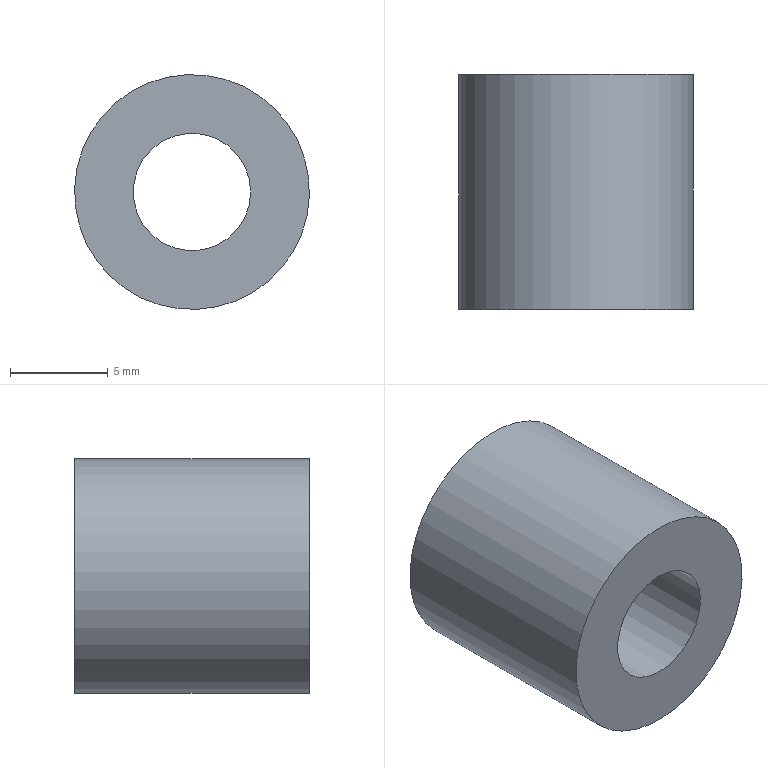Component | NX | LOCATING_BUSHING_2 | 1 solid | 4 faces | box 12 x 12 x 12 mm | volume 1018 mm3 | cylinder 2 | plane 2 | commonest cylinder face diameters 12 x1 6 x1
STEP:
#1=CARTESIAN_POINT('',(0.,0.,0.));
#2=DIRECTION('',(0.,0.,1.));
#3=DIRECTION('',(1.,0.,0.));
#4=AXIS2_PLACEMENT_3D('',#1,#2,#3);
#5=CARTESIAN_POINT('',(4.596,-12.,29.643));
#6=VERTEX_POINT('',#5);
#7=CARTESIAN_POINT('',(0.,-12.,33.5));
#8=DIRECTION('',(0.,-1.,0.));
#9=DIRECTION('',(0.766,0.,-0.6428));
#10=AXIS2_PLACEMENT_3D('',#7,#8,#9);
#11=CIRCLE('',#10,6.);
#12=CARTESIAN_POINT('',(0.,-12.,33.5));
#13=DIRECTION('',(0.,1.,0.));
#14=DIRECTION('',(0.6428,0.,0.766));
#15=AXIS2_PLACEMENT_3D('',#12,#13,#14);
#16=CYLINDRICAL_SURFACE('',#15,6.);
#17=CARTESIAN_POINT('',(7.854,0.));
#18=DIRECTION('',(-1.,0.));
#19=VECTOR('',#18,1.);
#20=LINE('',#17,#19);
#21=(GEOMETRIC_REPRESENTATION_CONTEXT(2)PARAMETRIC_REPRESENTATION_CONTEXT()REPRESENTATION_CONTEXT('',''));
#22=DEFINITIONAL_REPRESENTATION('',(#20),#21);
#23=PCURVE('',#16,#22);
#24=CARTESIAN_POINT('',(0.,-12.,33.5));
#25=DIRECTION('',(0.,-1.,0.));
#26=DIRECTION('',(-0.6428,0.,-0.766));
#27=AXIS2_PLACEMENT_3D('',#24,#25,#26);
#28=PLANE('',#27);
#29=CARTESIAN_POINT('',(0.,0.));
#30=DIRECTION('',(0.,1.));
#31=AXIS2_PLACEMENT_2D('',#29,#30);
#32=CIRCLE('',#31,6.);
#33=(GEOMETRIC_REPRESENTATION_CONTEXT(2)PARAMETRIC_REPRESENTATION_CONTEXT()REPRESENTATION_CONTEXT('',''));
#34=DEFINITIONAL_REPRESENTATION('',(#32),#33);
#35=PCURVE('',#28,#34);
#36=SURFACE_CURVE('',#11,(#23,#35),.PCURVE_S1.);
#37=EDGE_CURVE('',#6,#6,#36,.T.);
#38=ORIENTED_EDGE('',*,*,#37,.F.);
#39=CARTESIAN_POINT('',(4.596,0.,29.643));
#40=VERTEX_POINT('',#39);
#41=CARTESIAN_POINT('',(4.596,-12.,29.643));
#42=CARTESIAN_POINT('',(4.596,0.,29.643));
#43=B_SPLINE_CURVE_WITH_KNOTS('',1,(#41,#42),.UNSPECIFIED.,.F.,.F.,(2,2),(0.,12.),.PIECEWISE_BEZIER_KNOTS.);
#44=CARTESIAN_POINT('',(7.854,0.));
#45=DIRECTION('',(0.,1.));
#46=VECTOR('',#45,1.);
#47=LINE('',#44,#46);
#48=(GEOMETRIC_REPRESENTATION_CONTEXT(2)PARAMETRIC_REPRESENTATION_CONTEXT()REPRESENTATION_CONTEXT('',''));
#49=DEFINITIONAL_REPRESENTATION('',(#47),#48);
#50=PCURVE('',#16,#49);
#51=CARTESIAN_POINT('',(1.571,0.));
#52=DIRECTION('',(0.,1.));
#53=VECTOR('',#52,1.);
#54=LINE('',#51,#53);
#55=(GEOMETRIC_REPRESENTATION_CONTEXT(2)PARAMETRIC_REPRESENTATION_CONTEXT()REPRESENTATION_CONTEXT('',''));
#56=DEFINITIONAL_REPRESENTATION('',(#54),#55);
#57=PCURVE('',#16,#56);
#58=SEAM_CURVE('',#43,(#50,#57),.PCURVE_S1.);
#59=EDGE_CURVE('',#6,#40,#58,.T.);
#60=ORIENTED_EDGE('',*,*,#59,.T.);
#61=CARTESIAN_POINT('',(0.,0.,33.5));
#62=DIRECTION('',(0.,-1.,0.));
#63=DIRECTION('',(0.766,0.,-0.6428));
#64=AXIS2_PLACEMENT_3D('',#61,#62,#63);
#65=CIRCLE('',#64,6.);
#66=CARTESIAN_POINT('',(7.854,12.));
#67=DIRECTION('',(-1.,0.));
#68=VECTOR('',#67,1.);
#69=LINE('',#66,#68);
#70=(GEOMETRIC_REPRESENTATION_CONTEXT(2)PARAMETRIC_REPRESENTATION_CONTEXT()REPRESENTATION_CONTEXT('',''));
#71=DEFINITIONAL_REPRESENTATION('',(#69),#70);
#72=PCURVE('',#16,#71);
#73=CARTESIAN_POINT('',(0.,0.,33.5));
#74=DIRECTION('',(0.,-1.,0.));
#75=DIRECTION('',(-0.6428,0.,-0.766));
#76=AXIS2_PLACEMENT_3D('',#73,#74,#75);
#77=PLANE('',#76);
#78=CARTESIAN_POINT('',(0.,0.));
#79=DIRECTION('',(0.,1.));
#80=AXIS2_PLACEMENT_2D('',#78,#79);
#81=CIRCLE('',#80,6.);
#82=(GEOMETRIC_REPRESENTATION_CONTEXT(2)PARAMETRIC_REPRESENTATION_CONTEXT()REPRESENTATION_CONTEXT('',''));
#83=DEFINITIONAL_REPRESENTATION('',(#81),#82);
#84=PCURVE('',#77,#83);
#85=SURFACE_CURVE('',#65,(#72,#84),.PCURVE_S1.);
#86=EDGE_CURVE('',#40,#40,#85,.T.);
#87=ORIENTED_EDGE('',*,*,#86,.T.);
#88=ORIENTED_EDGE('',*,*,#59,.F.);
#89=EDGE_LOOP('',(#38,#60,#87,#88));
#90=FACE_BOUND('',#89,.T.);
#91=ADVANCED_FACE('',(#90),#16,.T.);
#92=CARTESIAN_POINT('',(2.298,-12.,31.572));
#93=VERTEX_POINT('',#92);
#94=CARTESIAN_POINT('',(0.,-12.,33.5));
#95=DIRECTION('',(0.,-1.,0.));
#96=DIRECTION('',(0.766,0.,-0.6428));
#97=AXIS2_PLACEMENT_3D('',#94,#95,#96);
#98=CIRCLE('',#97,3.);
#99=CARTESIAN_POINT('',(0.,-12.,33.5));
#100=DIRECTION('',(0.,1.,0.));
#101=DIRECTION('',(0.6428,0.,0.766));
#102=AXIS2_PLACEMENT_3D('',#99,#100,#101);
#103=CYLINDRICAL_SURFACE('',#102,3.);
#104=CARTESIAN_POINT('',(7.854,0.));
#105=DIRECTION('',(-1.,0.));
#106=VECTOR('',#105,1.);
#107=LINE('',#104,#106);
#108=(GEOMETRIC_REPRESENTATION_CONTEXT(2)PARAMETRIC_REPRESENTATION_CONTEXT()REPRESENTATION_CONTEXT('',''));
#109=DEFINITIONAL_REPRESENTATION('',(#107),#108);
#110=PCURVE('',#103,#109);
#111=CARTESIAN_POINT('',(0.,0.));
#112=DIRECTION('',(-0.,1.));
#113=AXIS2_PLACEMENT_2D('',#111,#112);
#114=CIRCLE('',#113,3.);
#115=(GEOMETRIC_REPRESENTATION_CONTEXT(2)PARAMETRIC_REPRESENTATION_CONTEXT()REPRESENTATION_CONTEXT('',''));
#116=DEFINITIONAL_REPRESENTATION('',(#114),#115);
#117=PCURVE('',#28,#116);
#118=SURFACE_CURVE('',#98,(#110,#117),.PCURVE_S1.);
#119=EDGE_CURVE('',#93,#93,#118,.T.);
#120=ORIENTED_EDGE('',*,*,#119,.F.);
#121=CARTESIAN_POINT('',(2.298,0.,31.572));
#122=VERTEX_POINT('',#121);
#123=CARTESIAN_POINT('',(2.298,-12.,31.572));
#124=CARTESIAN_POINT('',(2.298,0.,31.572));
#125=B_SPLINE_CURVE_WITH_KNOTS('',1,(#123,#124),.UNSPECIFIED.,.F.,.F.,(2,2),(0.,12.),.PIECEWISE_BEZIER_KNOTS.);
#126=CARTESIAN_POINT('',(7.854,0.));
#127=DIRECTION('',(0.,1.));
#128=VECTOR('',#127,1.);
#129=LINE('',#126,#128);
#130=(GEOMETRIC_REPRESENTATION_CONTEXT(2)PARAMETRIC_REPRESENTATION_CONTEXT()REPRESENTATION_CONTEXT('',''));
#131=DEFINITIONAL_REPRESENTATION('',(#129),#130);
#132=PCURVE('',#103,#131);
#133=CARTESIAN_POINT('',(1.571,0.));
#134=DIRECTION('',(0.,1.));
#135=VECTOR('',#134,1.);
#136=LINE('',#133,#135);
#137=(GEOMETRIC_REPRESENTATION_CONTEXT(2)PARAMETRIC_REPRESENTATION_CONTEXT()REPRESENTATION_CONTEXT('',''));
#138=DEFINITIONAL_REPRESENTATION('',(#136),#137);
#139=PCURVE('',#103,#138);
#140=SEAM_CURVE('',#125,(#132,#139),.PCURVE_S1.);
#141=EDGE_CURVE('',#93,#122,#140,.T.);
#142=ORIENTED_EDGE('',*,*,#141,.T.);
#143=CARTESIAN_POINT('',(0.,0.,33.5));
#144=DIRECTION('',(0.,-1.,0.));
#145=DIRECTION('',(0.766,0.,-0.6428));
#146=AXIS2_PLACEMENT_3D('',#143,#144,#145);
#147=CIRCLE('',#146,3.);
#148=CARTESIAN_POINT('',(7.854,12.));
#149=DIRECTION('',(-1.,0.));
#150=VECTOR('',#149,1.);
#151=LINE('',#148,#150);
#152=(GEOMETRIC_REPRESENTATION_CONTEXT(2)PARAMETRIC_REPRESENTATION_CONTEXT()REPRESENTATION_CONTEXT('',''));
#153=DEFINITIONAL_REPRESENTATION('',(#151),#152);
#154=PCURVE('',#103,#153);
#155=CARTESIAN_POINT('',(0.,0.));
#156=DIRECTION('',(-0.,1.));
#157=AXIS2_PLACEMENT_2D('',#155,#156);
#158=CIRCLE('',#157,3.);
#159=(GEOMETRIC_REPRESENTATION_CONTEXT(2)PARAMETRIC_REPRESENTATION_CONTEXT()REPRESENTATION_CONTEXT('',''));
#160=DEFINITIONAL_REPRESENTATION('',(#158),#159);
#161=PCURVE('',#77,#160);
#162=SURFACE_CURVE('',#147,(#154,#161),.PCURVE_S1.);
#163=EDGE_CURVE('',#122,#122,#162,.T.);
#164=ORIENTED_EDGE('',*,*,#163,.T.);
#165=ORIENTED_EDGE('',*,*,#141,.F.);
#166=EDGE_LOOP('',(#120,#142,#164,#165));
#167=FACE_BOUND('',#166,.F.);
#168=ADVANCED_FACE('',(#167),#103,.F.);
#169=ORIENTED_EDGE('',*,*,#37,.T.);
#170=EDGE_LOOP('',(#169));
#171=FACE_BOUND('',#170,.T.);
#172=ORIENTED_EDGE('',*,*,#119,.F.);
#173=EDGE_LOOP('',(#172));
#174=FACE_BOUND('',#173,.T.);
#175=ADVANCED_FACE('',(#171,#174),#28,.T.);
#176=ORIENTED_EDGE('',*,*,#86,.F.);
#177=EDGE_LOOP('',(#176));
#178=FACE_BOUND('',#177,.T.);
#179=ORIENTED_EDGE('',*,*,#163,.T.);
#180=EDGE_LOOP('',(#179));
#181=FACE_BOUND('',#180,.T.);
#182=ADVANCED_FACE('',(#178,#181),#77,.F.);
#183=CLOSED_SHELL('',(#91,#168,#175,#182));
#184=MANIFOLD_SOLID_BREP('',#183);
#185=(LENGTH_UNIT()NAMED_UNIT(*)SI_UNIT(.MILLI.,.METRE.));
#186=UNCERTAINTY_MEASURE_WITH_UNIT(LENGTH_MEASURE(0.00001),#185,'','');
#187=(NAMED_UNIT(*)PLANE_ANGLE_UNIT()SI_UNIT($,.RADIAN.));
#188=(NAMED_UNIT(*)SI_UNIT($,.STERADIAN.)SOLID_ANGLE_UNIT());
#189=(GEOMETRIC_REPRESENTATION_CONTEXT(3)GLOBAL_UNCERTAINTY_ASSIGNED_CONTEXT((#186))GLOBAL_UNIT_ASSIGNED_CONTEXT((#185,#187,#188))REPRESENTATION_CONTEXT('',''));
#190=ADVANCED_BREP_SHAPE_REPRESENTATION('',(#4,#184),#189);